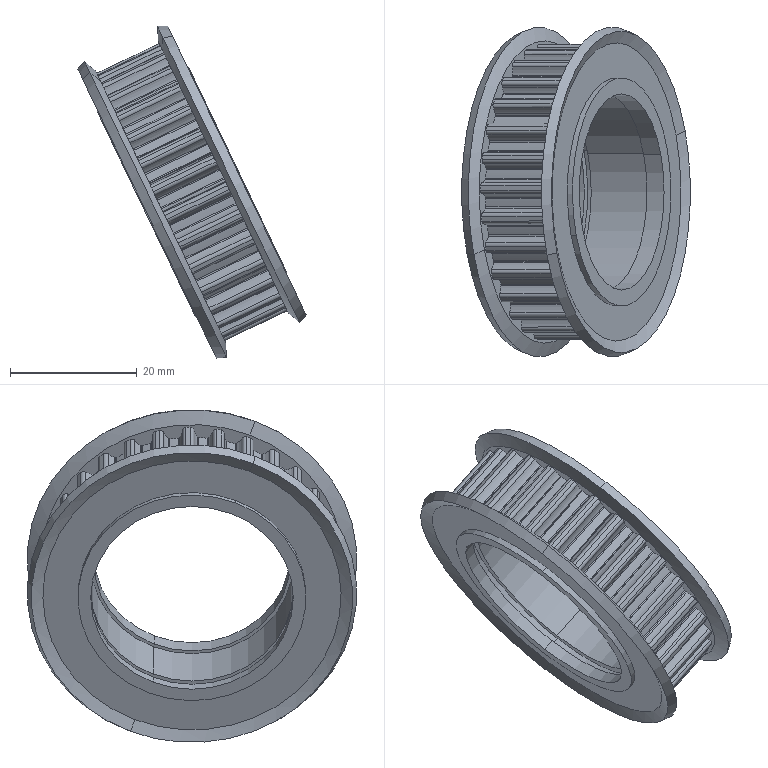Component | SolidWorks | AHTF30S5M100-1_AHTF30S5M100body-1 | 1 solid | 298 faces | volume 13038 mm3 | cylinder 277 | cone 12 | plane 9 | commonest cylinder face diameters 1.1 x72 0.5 x68 6.55 x64 46.79 x31 43.25 x30 36 x4 32 x4 34.4 x2